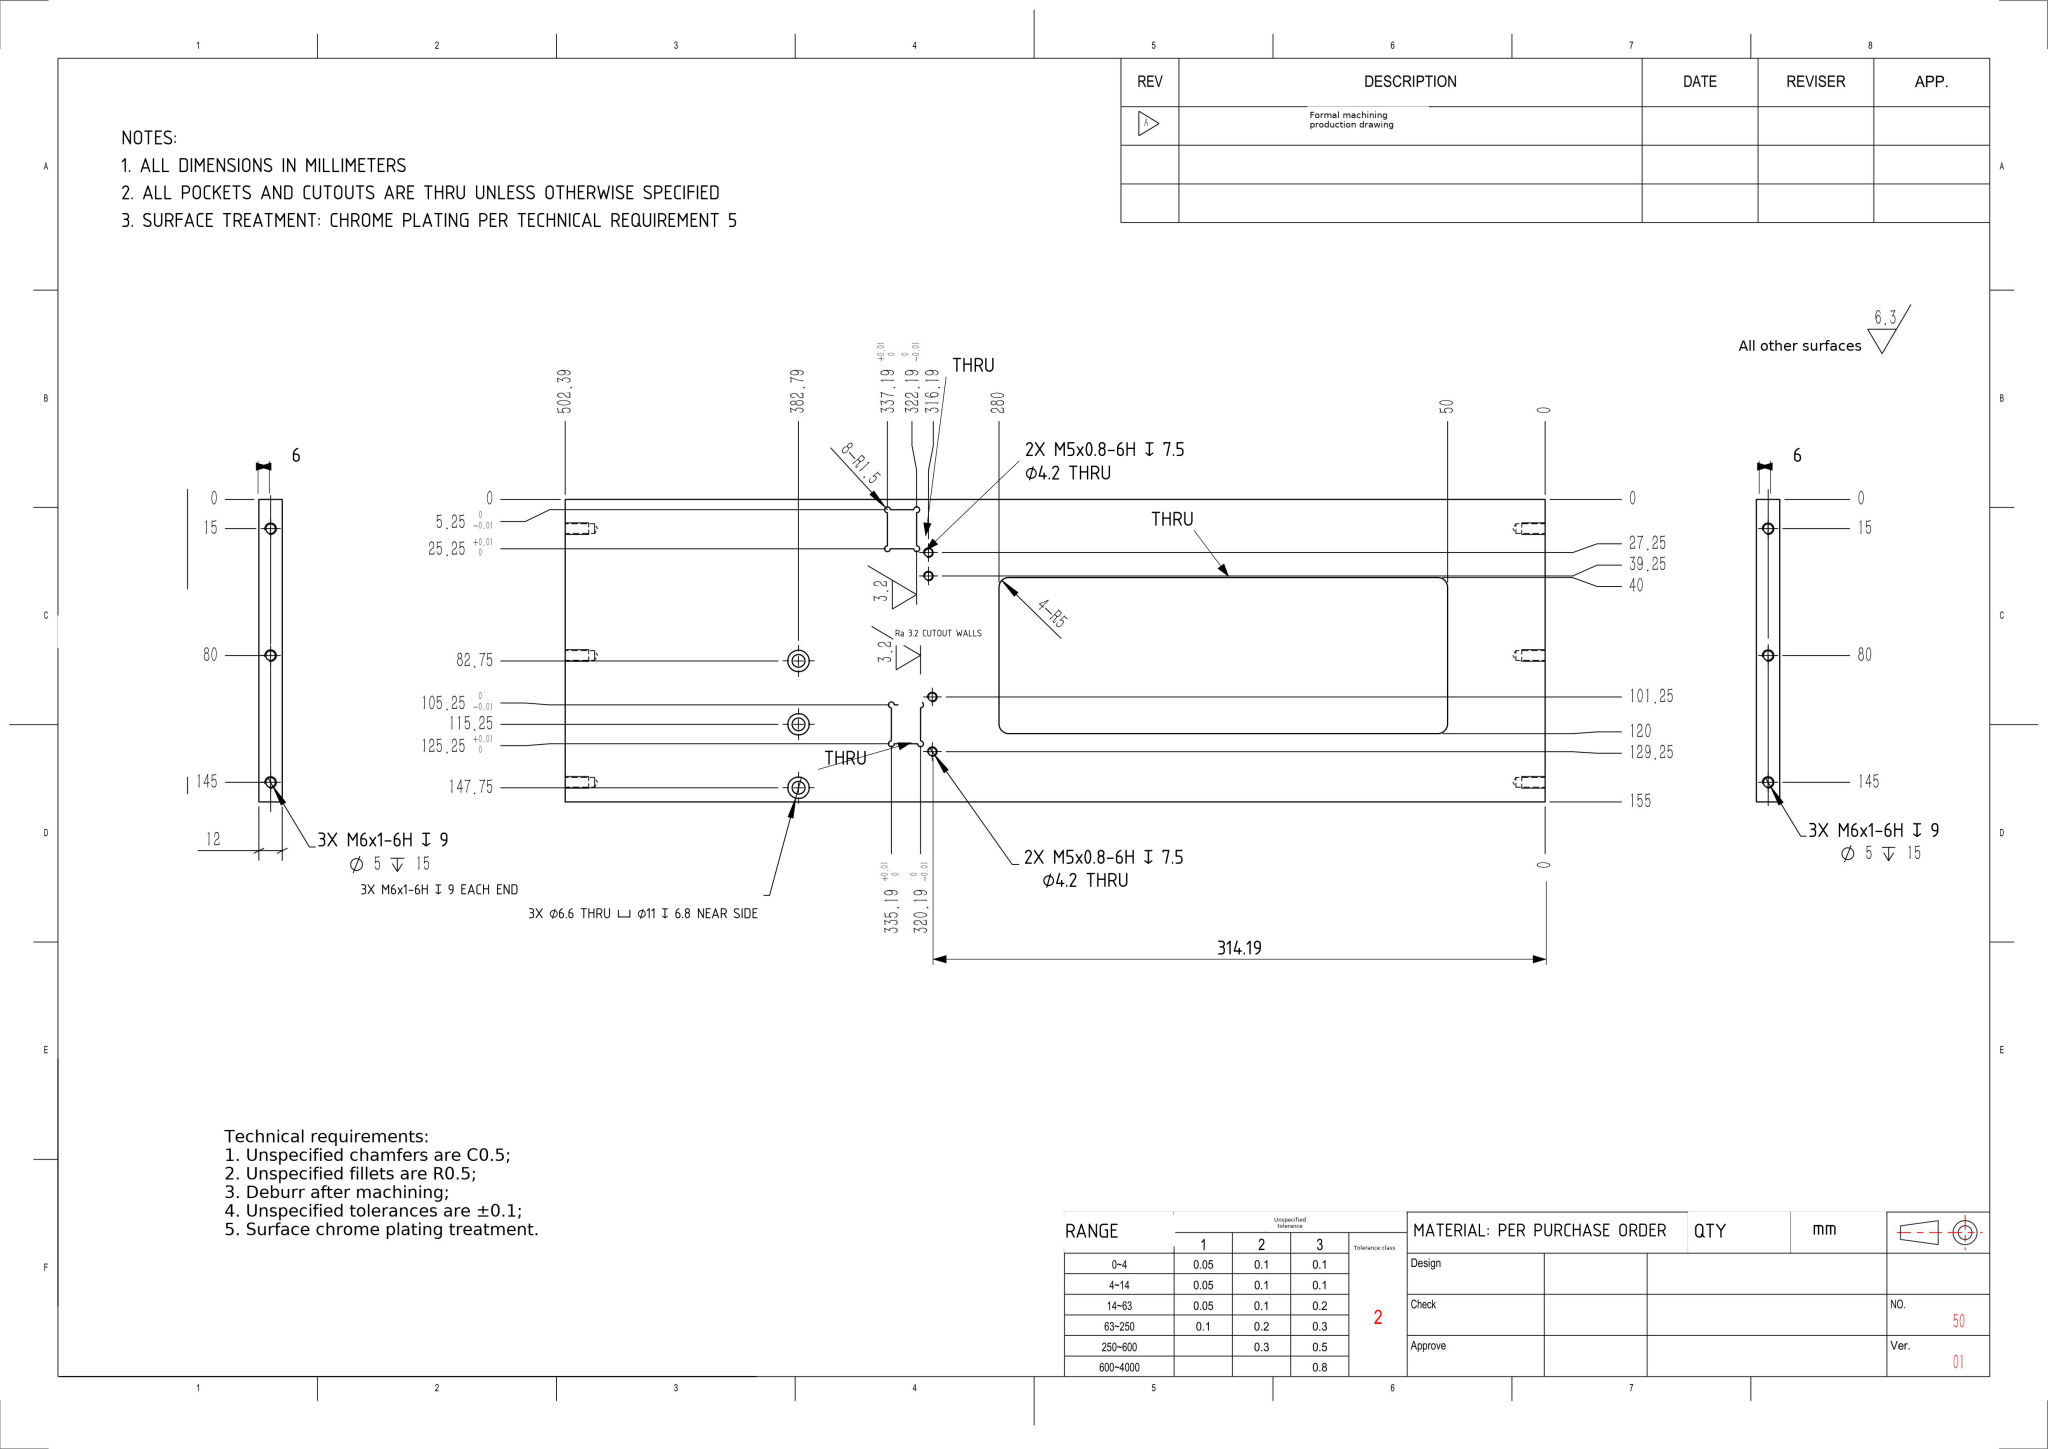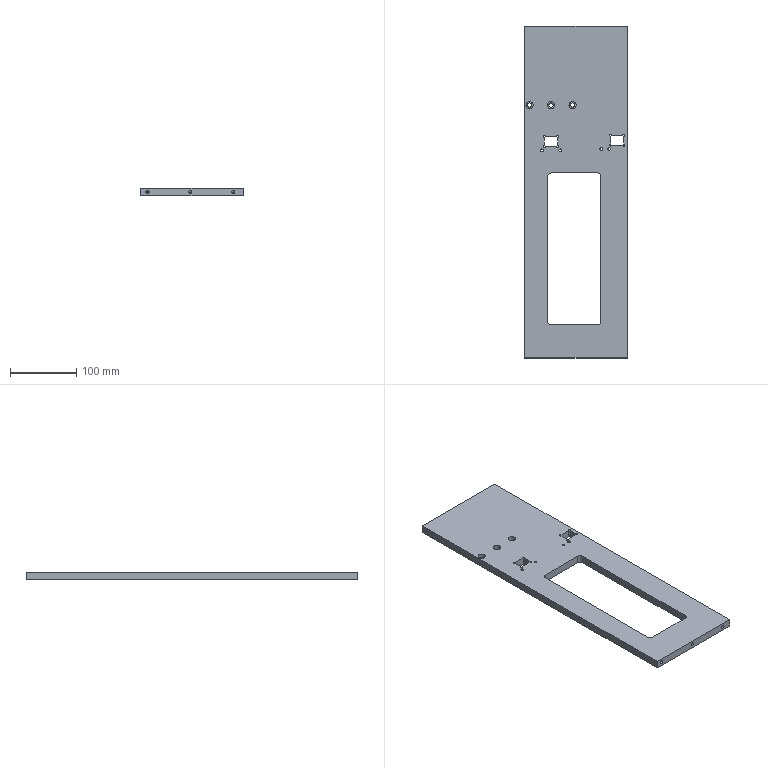Part | NX | mm | 1 solid | 81 faces | box 155 x 502.39 x 12 mm | volume 701230 mm3 | cylinder 48 | plane 21 | cone 12 | commonest cylinder face diameters 3 x12 5 x12 4.2 x8 11 x6 6.6 x6 10 x4